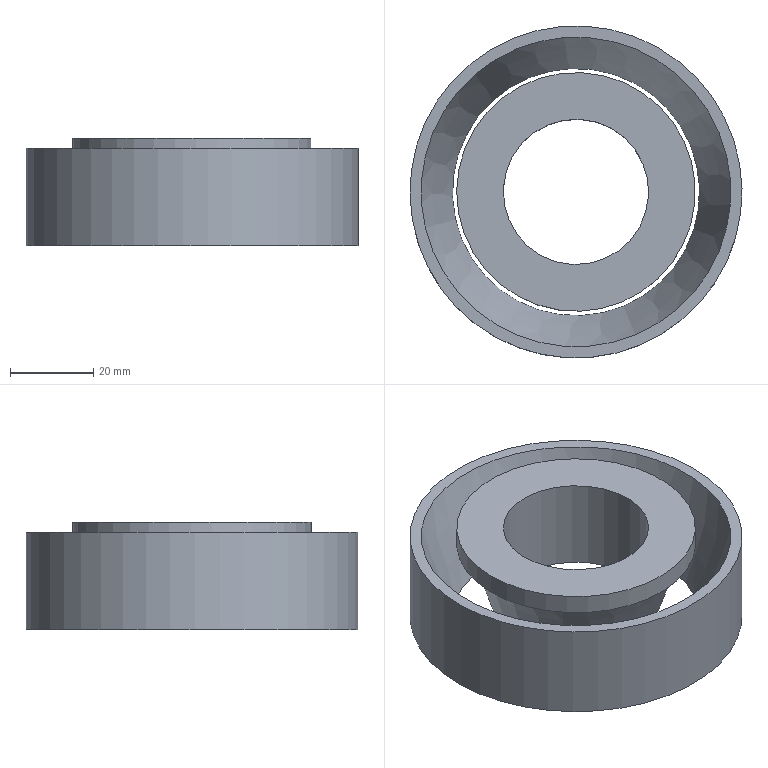Component | NX | GUNZIZHOUCHOU | 2 solids | 10 faces | box 80 x 80 x 26 mm | volume 55024 mm3 | plane 5 | cylinder 3 | cone 2 | commonest cylinder face diameters 35 x1 57.5 x1 80 x1
STEP:
#1=CARTESIAN_POINT('',(0.,0.,0.));
#2=DIRECTION('',(0.,0.,1.));
#3=DIRECTION('',(1.,0.,0.));
#4=AXIS2_PLACEMENT_3D('',#1,#2,#3);
#5=CARTESIAN_POINT('',(6.703,-16.165,0.45));
#6=VERTEX_POINT('',#5);
#7=CARTESIAN_POINT('',(0.,0.,0.45));
#8=DIRECTION('',(0.,0.,1.));
#9=DIRECTION('',(0.383,-0.9237,0.));
#10=AXIS2_PLACEMENT_3D('',#7,#8,#9);
#11=CIRCLE('',#10,17.5);
#12=CARTESIAN_POINT('',(18.43,7.643,0.45));
#13=DIRECTION('',(0.,0.,-1.));
#14=DIRECTION('',(-0.383,0.9237,0.));
#15=AXIS2_PLACEMENT_3D('',#12,#13,#14);
#16=PLANE('',#15);
#17=CARTESIAN_POINT('',(-17.5,-19.952));
#18=CARTESIAN_POINT('',(-17.5,10.359));
#19=CARTESIAN_POINT('',(8.75,-4.797));
#20=CARTESIAN_POINT('',(35.,-19.952));
#21=CARTESIAN_POINT('',(8.75,-35.107));
#22=CARTESIAN_POINT('',(-17.5,-50.263));
#23=CARTESIAN_POINT('',(-17.5,-19.952));
#24=(BOUNDED_CURVE()B_SPLINE_CURVE(2,(#17,#18,#19,#20,#21,#22,#23),.UNSPECIFIED.,.T.,.F.)B_SPLINE_CURVE_WITH_KNOTS((1,2,2,2,2,1),(-2.094,0.,2.094,4.189,6.283,8.378),.UNSPECIFIED.)CURVE()GEOMETRIC_REPRESENTATION_ITEM()RATIONAL_B_SPLINE_CURVE((1.,0.5,1.,0.5,1.,0.5,1.))REPRESENTATION_ITEM(''));
#25=(GEOMETRIC_REPRESENTATION_CONTEXT(2)PARAMETRIC_REPRESENTATION_CONTEXT()REPRESENTATION_CONTEXT('',''));
#26=DEFINITIONAL_REPRESENTATION('',(#24),#25);
#27=PCURVE('',#16,#26);
#28=CARTESIAN_POINT('',(0.,0.,23.));
#29=DIRECTION('',(0.,0.,1.));
#30=DIRECTION('',(0.383,-0.9237,0.));
#31=AXIS2_PLACEMENT_3D('',#28,#29,#30);
#32=CYLINDRICAL_SURFACE('',#31,17.5);
#33=CARTESIAN_POINT('',(0.,-22.55));
#34=DIRECTION('',(1.,0.));
#35=VECTOR('',#34,1.);
#36=LINE('',#33,#35);
#37=(GEOMETRIC_REPRESENTATION_CONTEXT(2)PARAMETRIC_REPRESENTATION_CONTEXT()REPRESENTATION_CONTEXT('',''));
#38=DEFINITIONAL_REPRESENTATION('',(#36),#37);
#39=PCURVE('',#32,#38);
#40=SURFACE_CURVE('',#11,(#27,#39),.PCURVE_S1.);
#41=EDGE_CURVE('',#6,#6,#40,.T.);
#42=ORIENTED_EDGE('',*,*,#41,.T.);
#43=EDGE_LOOP('',(#42));
#44=FACE_BOUND('',#43,.T.);
#45=CARTESIAN_POINT('',(7.643,-18.43,0.45));
#46=VERTEX_POINT('',#45);
#47=CARTESIAN_POINT('',(0.,0.,0.45));
#48=DIRECTION('',(0.,0.,1.));
#49=DIRECTION('',(0.383,-0.9237,0.));
#50=AXIS2_PLACEMENT_3D('',#47,#48,#49);
#51=CIRCLE('',#50,19.952);
#52=CARTESIAN_POINT('',(-19.952,-19.952));
#53=CARTESIAN_POINT('',(-19.952,14.606));
#54=CARTESIAN_POINT('',(9.976,-2.673));
#55=CARTESIAN_POINT('',(39.904,-19.952));
#56=CARTESIAN_POINT('',(9.976,-37.231));
#57=CARTESIAN_POINT('',(-19.952,-54.51));
#58=CARTESIAN_POINT('',(-19.952,-19.952));
#59=(BOUNDED_CURVE()B_SPLINE_CURVE(2,(#52,#53,#54,#55,#56,#57,#58),.UNSPECIFIED.,.T.,.F.)B_SPLINE_CURVE_WITH_KNOTS((1,2,2,2,2,1),(-2.094,0.,2.094,4.189,6.283,8.378),.UNSPECIFIED.)CURVE()GEOMETRIC_REPRESENTATION_ITEM()RATIONAL_B_SPLINE_CURVE((1.,0.5,1.,0.5,1.,0.5,1.))REPRESENTATION_ITEM(''));
#60=(GEOMETRIC_REPRESENTATION_CONTEXT(2)PARAMETRIC_REPRESENTATION_CONTEXT()REPRESENTATION_CONTEXT('',''));
#61=DEFINITIONAL_REPRESENTATION('',(#59),#60);
#62=PCURVE('',#16,#61);
#63=CARTESIAN_POINT('',(0.,0.,18.25));
#64=DIRECTION('',(0.,0.,1.));
#65=DIRECTION('',(0.383,-0.9237,0.));
#66=AXIS2_PLACEMENT_3D('',#63,#64,#65);
#67=CONICAL_SURFACE('',#66,25.952,0.3251);
#68=CARTESIAN_POINT('',(0.,-17.8));
#69=DIRECTION('',(1.,0.));
#70=VECTOR('',#69,1.);
#71=LINE('',#68,#70);
#72=(GEOMETRIC_REPRESENTATION_CONTEXT(2)PARAMETRIC_REPRESENTATION_CONTEXT()REPRESENTATION_CONTEXT('',''));
#73=DEFINITIONAL_REPRESENTATION('',(#71),#72);
#74=PCURVE('',#67,#73);
#75=SURFACE_CURVE('',#51,(#62,#74),.PCURVE_S1.);
#76=EDGE_CURVE('',#46,#46,#75,.T.);
#77=ORIENTED_EDGE('',*,*,#76,.F.);
#78=EDGE_LOOP('',(#77));
#79=FACE_BOUND('',#78,.T.);
#80=ADVANCED_FACE('',(#44,#79),#16,.T.);
#81=CARTESIAN_POINT('',(6.703,-16.165,23.));
#82=VERTEX_POINT('',#81);
#83=CARTESIAN_POINT('',(0.,0.,23.));
#84=DIRECTION('',(0.,0.,1.));
#85=DIRECTION('',(0.383,-0.9237,0.));
#86=AXIS2_PLACEMENT_3D('',#83,#84,#85);
#87=CIRCLE('',#86,17.5);
#88=CARTESIAN_POINT('',(0.,0.));
#89=DIRECTION('',(1.,0.));
#90=VECTOR('',#89,1.);
#91=LINE('',#88,#90);
#92=(GEOMETRIC_REPRESENTATION_CONTEXT(2)PARAMETRIC_REPRESENTATION_CONTEXT()REPRESENTATION_CONTEXT('',''));
#93=DEFINITIONAL_REPRESENTATION('',(#91),#92);
#94=PCURVE('',#32,#93);
#95=CARTESIAN_POINT('',(16.165,6.703,23.));
#96=DIRECTION('',(0.,0.,1.));
#97=DIRECTION('',(0.383,-0.9237,0.));
#98=AXIS2_PLACEMENT_3D('',#95,#96,#97);
#99=PLANE('',#98);
#100=CARTESIAN_POINT('',(-0.,-17.5));
#101=DIRECTION('',(1.,0.));
#102=AXIS2_PLACEMENT_2D('',#100,#101);
#103=CIRCLE('',#102,17.5);
#104=(GEOMETRIC_REPRESENTATION_CONTEXT(2)PARAMETRIC_REPRESENTATION_CONTEXT()REPRESENTATION_CONTEXT('',''));
#105=DEFINITIONAL_REPRESENTATION('',(#103),#104);
#106=PCURVE('',#99,#105);
#107=SURFACE_CURVE('',#87,(#94,#106),.PCURVE_S1.);
#108=EDGE_CURVE('',#82,#82,#107,.T.);
#109=ORIENTED_EDGE('',*,*,#108,.F.);
#110=CARTESIAN_POINT('',(6.703,-16.165,0.45));
#111=CARTESIAN_POINT('',(6.703,-16.165,23.));
#112=B_SPLINE_CURVE_WITH_KNOTS('',1,(#110,#111),.UNSPECIFIED.,.F.,.F.,(2,2),(-22.55,0.),.PIECEWISE_BEZIER_KNOTS.);
#113=CARTESIAN_POINT('',(0.,0.));
#114=DIRECTION('',(0.,1.));
#115=VECTOR('',#114,1.);
#116=LINE('',#113,#115);
#117=(GEOMETRIC_REPRESENTATION_CONTEXT(2)PARAMETRIC_REPRESENTATION_CONTEXT()REPRESENTATION_CONTEXT('',''));
#118=DEFINITIONAL_REPRESENTATION('',(#116),#117);
#119=PCURVE('',#32,#118);
#120=CARTESIAN_POINT('',(6.283,0.));
#121=DIRECTION('',(0.,1.));
#122=VECTOR('',#121,1.);
#123=LINE('',#120,#122);
#124=(GEOMETRIC_REPRESENTATION_CONTEXT(2)PARAMETRIC_REPRESENTATION_CONTEXT()REPRESENTATION_CONTEXT('',''));
#125=DEFINITIONAL_REPRESENTATION('',(#123),#124);
#126=PCURVE('',#32,#125);
#127=SEAM_CURVE('',#112,(#119,#126),.PCURVE_S1.);
#128=EDGE_CURVE('',#6,#82,#127,.T.);
#129=ORIENTED_EDGE('',*,*,#128,.F.);
#130=ORIENTED_EDGE('',*,*,#41,.T.);
#131=ORIENTED_EDGE('',*,*,#128,.T.);
#132=EDGE_LOOP('',(#109,#129,#130,#131));
#133=FACE_BOUND('',#132,.F.);
#134=ADVANCED_FACE('',(#133),#32,.F.);
#135=CARTESIAN_POINT('',(11.013,-26.557,23.));
#136=VERTEX_POINT('',#135);
#137=CARTESIAN_POINT('',(0.,0.,23.));
#138=DIRECTION('',(0.,0.,1.));
#139=DIRECTION('',(0.383,-0.9237,0.));
#140=AXIS2_PLACEMENT_3D('',#137,#138,#139);
#141=CIRCLE('',#140,28.75);
#142=CARTESIAN_POINT('',(-0.,-17.5));
#143=DIRECTION('',(1.,0.));
#144=AXIS2_PLACEMENT_2D('',#142,#143);
#145=CIRCLE('',#144,28.75);
#146=(GEOMETRIC_REPRESENTATION_CONTEXT(2)PARAMETRIC_REPRESENTATION_CONTEXT()REPRESENTATION_CONTEXT('',''));
#147=DEFINITIONAL_REPRESENTATION('',(#145),#146);
#148=PCURVE('',#99,#147);
#149=CARTESIAN_POINT('',(0.,0.,23.));
#150=DIRECTION('',(0.,0.,1.));
#151=DIRECTION('',(0.383,-0.9237,0.));
#152=AXIS2_PLACEMENT_3D('',#149,#150,#151);
#153=CYLINDRICAL_SURFACE('',#152,28.75);
#154=CARTESIAN_POINT('',(0.,0.));
#155=DIRECTION('',(1.,0.));
#156=VECTOR('',#155,1.);
#157=LINE('',#154,#156);
#158=(GEOMETRIC_REPRESENTATION_CONTEXT(2)PARAMETRIC_REPRESENTATION_CONTEXT()REPRESENTATION_CONTEXT('',''));
#159=DEFINITIONAL_REPRESENTATION('',(#157),#158);
#160=PCURVE('',#153,#159);
#161=SURFACE_CURVE('',#141,(#148,#160),.PCURVE_S1.);
#162=EDGE_CURVE('',#136,#136,#161,.T.);
#163=ORIENTED_EDGE('',*,*,#162,.T.);
#164=EDGE_LOOP('',(#163));
#165=FACE_BOUND('',#164,.T.);
#166=ORIENTED_EDGE('',*,*,#108,.F.);
#167=EDGE_LOOP('',(#166));
#168=FACE_BOUND('',#167,.T.);
#169=ADVANCED_FACE('',(#165,#168),#99,.T.);
#170=CARTESIAN_POINT('',(11.013,-26.557,18.25));
#171=VERTEX_POINT('',#170);
#172=CARTESIAN_POINT('',(0.,0.,18.25));
#173=DIRECTION('',(0.,0.,1.));
#174=DIRECTION('',(0.383,-0.9237,0.));
#175=AXIS2_PLACEMENT_3D('',#172,#173,#174);
#176=CIRCLE('',#175,28.75);
#177=CARTESIAN_POINT('',(0.,-4.75));
#178=DIRECTION('',(1.,0.));
#179=VECTOR('',#178,1.);
#180=LINE('',#177,#179);
#181=(GEOMETRIC_REPRESENTATION_CONTEXT(2)PARAMETRIC_REPRESENTATION_CONTEXT()REPRESENTATION_CONTEXT('',''));
#182=DEFINITIONAL_REPRESENTATION('',(#180),#181);
#183=PCURVE('',#153,#182);
#184=CARTESIAN_POINT('',(26.557,11.013,18.25));
#185=DIRECTION('',(0.,0.,-1.));
#186=DIRECTION('',(-0.383,0.9237,0.));
#187=AXIS2_PLACEMENT_3D('',#184,#185,#186);
#188=PLANE('',#187);
#189=CARTESIAN_POINT('',(-28.75,-28.75));
#190=CARTESIAN_POINT('',(-28.75,21.046));
#191=CARTESIAN_POINT('',(14.375,-3.852));
#192=CARTESIAN_POINT('',(57.5,-28.75));
#193=CARTESIAN_POINT('',(14.375,-53.648));
#194=CARTESIAN_POINT('',(-28.75,-78.546));
#195=CARTESIAN_POINT('',(-28.75,-28.75));
#196=(BOUNDED_CURVE()B_SPLINE_CURVE(2,(#189,#190,#191,#192,#193,#194,#195),.UNSPECIFIED.,.T.,.F.)B_SPLINE_CURVE_WITH_KNOTS((1,2,2,2,2,1),(-2.094,0.,2.094,4.189,6.283,8.378),.UNSPECIFIED.)CURVE()GEOMETRIC_REPRESENTATION_ITEM()RATIONAL_B_SPLINE_CURVE((1.,0.5,1.,0.5,1.,0.5,1.))REPRESENTATION_ITEM(''));
#197=(GEOMETRIC_REPRESENTATION_CONTEXT(2)PARAMETRIC_REPRESENTATION_CONTEXT()REPRESENTATION_CONTEXT('',''));
#198=DEFINITIONAL_REPRESENTATION('',(#196),#197);
#199=PCURVE('',#188,#198);
#200=SURFACE_CURVE('',#176,(#183,#199),.PCURVE_S1.);
#201=EDGE_CURVE('',#171,#171,#200,.T.);
#202=ORIENTED_EDGE('',*,*,#201,.T.);
#203=CARTESIAN_POINT('',(11.013,-26.557,18.25));
#204=CARTESIAN_POINT('',(11.013,-26.557,23.));
#205=B_SPLINE_CURVE_WITH_KNOTS('',1,(#203,#204),.UNSPECIFIED.,.F.,.F.,(2,2),(-4.75,0.),.PIECEWISE_BEZIER_KNOTS.);
#206=CARTESIAN_POINT('',(6.283,0.));
#207=DIRECTION('',(0.,1.));
#208=VECTOR('',#207,1.);
#209=LINE('',#206,#208);
#210=(GEOMETRIC_REPRESENTATION_CONTEXT(2)PARAMETRIC_REPRESENTATION_CONTEXT()REPRESENTATION_CONTEXT('',''));
#211=DEFINITIONAL_REPRESENTATION('',(#209),#210);
#212=PCURVE('',#153,#211);
#213=CARTESIAN_POINT('',(0.,0.));
#214=DIRECTION('',(0.,1.));
#215=VECTOR('',#214,1.);
#216=LINE('',#213,#215);
#217=(GEOMETRIC_REPRESENTATION_CONTEXT(2)PARAMETRIC_REPRESENTATION_CONTEXT()REPRESENTATION_CONTEXT('',''));
#218=DEFINITIONAL_REPRESENTATION('',(#216),#217);
#219=PCURVE('',#153,#218);
#220=SEAM_CURVE('',#205,(#212,#219),.PCURVE_S1.);
#221=EDGE_CURVE('',#171,#136,#220,.T.);
#222=ORIENTED_EDGE('',*,*,#221,.T.);
#223=ORIENTED_EDGE('',*,*,#162,.F.);
#224=ORIENTED_EDGE('',*,*,#221,.F.);
#225=EDGE_LOOP('',(#202,#222,#223,#224));
#226=FACE_BOUND('',#225,.T.);
#227=ADVANCED_FACE('',(#226),#153,.T.);
#228=CARTESIAN_POINT('',(9.941,-23.973,18.25));
#229=VERTEX_POINT('',#228);
#230=CARTESIAN_POINT('',(0.,0.,18.25));
#231=DIRECTION('',(0.,0.,1.));
#232=DIRECTION('',(0.383,-0.9237,0.));
#233=AXIS2_PLACEMENT_3D('',#230,#231,#232);
#234=CIRCLE('',#233,25.952);
#235=CARTESIAN_POINT('',(-25.952,-28.75));
#236=CARTESIAN_POINT('',(-25.952,16.2));
#237=CARTESIAN_POINT('',(12.976,-6.275));
#238=CARTESIAN_POINT('',(51.904,-28.75));
#239=CARTESIAN_POINT('',(12.976,-51.225));
#240=CARTESIAN_POINT('',(-25.952,-73.7));
#241=CARTESIAN_POINT('',(-25.952,-28.75));
#242=(BOUNDED_CURVE()B_SPLINE_CURVE(2,(#235,#236,#237,#238,#239,#240,#241),.UNSPECIFIED.,.T.,.F.)B_SPLINE_CURVE_WITH_KNOTS((1,2,2,2,2,1),(-2.094,0.,2.094,4.189,6.283,8.378),.UNSPECIFIED.)CURVE()GEOMETRIC_REPRESENTATION_ITEM()RATIONAL_B_SPLINE_CURVE((1.,0.5,1.,0.5,1.,0.5,1.))REPRESENTATION_ITEM(''));
#243=(GEOMETRIC_REPRESENTATION_CONTEXT(2)PARAMETRIC_REPRESENTATION_CONTEXT()REPRESENTATION_CONTEXT('',''));
#244=DEFINITIONAL_REPRESENTATION('',(#242),#243);
#245=PCURVE('',#188,#244);
#246=CARTESIAN_POINT('',(0.,0.));
#247=DIRECTION('',(1.,-0.));
#248=VECTOR('',#247,1.);
#249=LINE('',#246,#248);
#250=(GEOMETRIC_REPRESENTATION_CONTEXT(2)PARAMETRIC_REPRESENTATION_CONTEXT()REPRESENTATION_CONTEXT('',''));
#251=DEFINITIONAL_REPRESENTATION('',(#249),#250);
#252=PCURVE('',#67,#251);
#253=SURFACE_CURVE('',#234,(#245,#252),.PCURVE_S1.);
#254=EDGE_CURVE('',#229,#229,#253,.T.);
#255=ORIENTED_EDGE('',*,*,#254,.T.);
#256=EDGE_LOOP('',(#255));
#257=FACE_BOUND('',#256,.T.);
#258=ORIENTED_EDGE('',*,*,#201,.F.);
#259=EDGE_LOOP('',(#258));
#260=FACE_BOUND('',#259,.T.);
#261=ADVANCED_FACE('',(#257,#260),#188,.T.);
#262=ORIENTED_EDGE('',*,*,#76,.T.);
#263=CARTESIAN_POINT('',(7.643,-18.43,0.45));
#264=CARTESIAN_POINT('',(9.941,-23.973,18.25));
#265=B_SPLINE_CURVE_WITH_KNOTS('',1,(#263,#264),.UNSPECIFIED.,.F.,.F.,(2,2),(-18.784,0.),.PIECEWISE_BEZIER_KNOTS.);
#266=CARTESIAN_POINT('',(6.283,0.));
#267=DIRECTION('',(0.,1.));
#268=VECTOR('',#267,1.);
#269=LINE('',#266,#268);
#270=(GEOMETRIC_REPRESENTATION_CONTEXT(2)PARAMETRIC_REPRESENTATION_CONTEXT()REPRESENTATION_CONTEXT('',''));
#271=DEFINITIONAL_REPRESENTATION('',(#269),#270);
#272=PCURVE('',#67,#271);
#273=CARTESIAN_POINT('',(0.,0.));
#274=DIRECTION('',(0.,1.));
#275=VECTOR('',#274,1.);
#276=LINE('',#273,#275);
#277=(GEOMETRIC_REPRESENTATION_CONTEXT(2)PARAMETRIC_REPRESENTATION_CONTEXT()REPRESENTATION_CONTEXT('',''));
#278=DEFINITIONAL_REPRESENTATION('',(#276),#277);
#279=PCURVE('',#67,#278);
#280=SEAM_CURVE('',#265,(#272,#279),.PCURVE_S1.);
#281=EDGE_CURVE('',#46,#229,#280,.T.);
#282=ORIENTED_EDGE('',*,*,#281,.T.);
#283=ORIENTED_EDGE('',*,*,#254,.F.);
#284=ORIENTED_EDGE('',*,*,#281,.F.);
#285=EDGE_LOOP('',(#262,#282,#283,#284));
#286=FACE_BOUND('',#285,.T.);
#287=ADVANCED_FACE('',(#286),#67,.T.);
#288=CLOSED_SHELL('',(#80,#134,#169,#227,#261,#287));
#289=MANIFOLD_SOLID_BREP('',#288);
#290=(LENGTH_UNIT()NAMED_UNIT(*)SI_UNIT(.MILLI.,.METRE.));
#291=UNCERTAINTY_MEASURE_WITH_UNIT(LENGTH_MEASURE(0.00001),#290,'','');
#292=(NAMED_UNIT(*)PLANE_ANGLE_UNIT()SI_UNIT($,.RADIAN.));
#293=(NAMED_UNIT(*)SI_UNIT($,.STERADIAN.)SOLID_ANGLE_UNIT());
#294=(GEOMETRIC_REPRESENTATION_CONTEXT(3)GLOBAL_UNCERTAINTY_ASSIGNED_CONTEXT((#291))GLOBAL_UNIT_ASSIGNED_CONTEXT((#290,#292,#293))REPRESENTATION_CONTEXT('',''));
#295=ADVANCED_BREP_SHAPE_REPRESENTATION('',(#4,#289),#294);
#296=CARTESIAN_POINT('',(0.,0.,0.));
#297=DIRECTION('',(0.,0.,1.));
#298=DIRECTION('',(1.,0.,0.));
#299=AXIS2_PLACEMENT_3D('',#296,#297,#298);
#300=CARTESIAN_POINT('',(0.,0.,0.));
#301=DIRECTION('',(0.,0.,1.));
#302=DIRECTION('',(1.,0.,0.));
#303=AXIS2_PLACEMENT_3D('',#300,#301,#302);
#304=(LENGTH_UNIT()NAMED_UNIT(*)SI_UNIT(.MILLI.,.METRE.));
#305=UNCERTAINTY_MEASURE_WITH_UNIT(LENGTH_MEASURE(0.00001),#304,'','');
#306=(NAMED_UNIT(*)PLANE_ANGLE_UNIT()SI_UNIT($,.RADIAN.));
#307=(NAMED_UNIT(*)SI_UNIT($,.STERADIAN.)SOLID_ANGLE_UNIT());
#308=(GEOMETRIC_REPRESENTATION_CONTEXT(3)GLOBAL_UNCERTAINTY_ASSIGNED_CONTEXT((#305))GLOBAL_UNIT_ASSIGNED_CONTEXT((#304,#306,#307))REPRESENTATION_CONTEXT('',''));
#309=SHAPE_REPRESENTATION('',(#4,#299,#303),#308);
#310=ITEM_DEFINED_TRANSFORMATION('','',#4,#299);
#311=(REPRESENTATION_RELATIONSHIP('','',#295,#309)REPRESENTATION_RELATIONSHIP_WITH_TRANSFORMATION(#310)SHAPE_REPRESENTATION_RELATIONSHIP());
#312=CARTESIAN_POINT('',(15.322,-36.949,20.5));
#313=VERTEX_POINT('',#312);
#314=CARTESIAN_POINT('',(0.,0.,20.5));
#315=DIRECTION('',(0.,0.,1.));
#316=DIRECTION('',(0.383,-0.9237,0.));
#317=AXIS2_PLACEMENT_3D('',#314,#315,#316);
#318=CIRCLE('',#317,40.);
#319=CARTESIAN_POINT('',(0.,0.,23.));
#320=DIRECTION('',(0.,0.,1.));
#321=DIRECTION('',(0.383,-0.9237,0.));
#322=AXIS2_PLACEMENT_3D('',#319,#320,#321);
#323=CYLINDRICAL_SURFACE('',#322,40.);
#324=CARTESIAN_POINT('',(0.,-2.5));
#325=DIRECTION('',(1.,0.));
#326=VECTOR('',#325,1.);
#327=LINE('',#324,#326);
#328=(GEOMETRIC_REPRESENTATION_CONTEXT(2)PARAMETRIC_REPRESENTATION_CONTEXT()REPRESENTATION_CONTEXT('',''));
#329=DEFINITIONAL_REPRESENTATION('',(#327),#328);
#330=PCURVE('',#323,#329);
#331=CARTESIAN_POINT('',(-15.322,36.949,20.5));
#332=DIRECTION('',(0.,0.,-1.));
#333=DIRECTION('',(-0.383,0.9237,0.));
#334=AXIS2_PLACEMENT_3D('',#331,#332,#333);
#335=PLANE('',#334);
#336=CARTESIAN_POINT('',(-80.,-0.));
#337=CARTESIAN_POINT('',(-80.,69.282));
#338=CARTESIAN_POINT('',(-20.,34.641));
#339=CARTESIAN_POINT('',(40.,-0.));
#340=CARTESIAN_POINT('',(-20.,-34.641));
#341=CARTESIAN_POINT('',(-80.,-69.282));
#342=CARTESIAN_POINT('',(-80.,-0.));
#343=(BOUNDED_CURVE()B_SPLINE_CURVE(2,(#336,#337,#338,#339,#340,#341,#342),.UNSPECIFIED.,.T.,.F.)B_SPLINE_CURVE_WITH_KNOTS((1,2,2,2,2,1),(-2.094,0.,2.094,4.189,6.283,8.378),.UNSPECIFIED.)CURVE()GEOMETRIC_REPRESENTATION_ITEM()RATIONAL_B_SPLINE_CURVE((1.,0.5,1.,0.5,1.,0.5,1.))REPRESENTATION_ITEM(''));
#344=(GEOMETRIC_REPRESENTATION_CONTEXT(2)PARAMETRIC_REPRESENTATION_CONTEXT()REPRESENTATION_CONTEXT('',''));
#345=DEFINITIONAL_REPRESENTATION('',(#343),#344);
#346=PCURVE('',#335,#345);
#347=SURFACE_CURVE('',#318,(#330,#346),.PCURVE_S1.);
#348=EDGE_CURVE('',#313,#313,#347,.T.);
#349=ORIENTED_EDGE('',*,*,#348,.F.);
#350=CARTESIAN_POINT('',(15.322,-36.949,-3.));
#351=VERTEX_POINT('',#350);
#352=CARTESIAN_POINT('',(15.322,-36.949,-3.));
#353=CARTESIAN_POINT('',(15.322,-36.949,20.5));
#354=B_SPLINE_CURVE_WITH_KNOTS('',1,(#352,#353),.UNSPECIFIED.,.F.,.F.,(2,2),(-26.,-2.5),.PIECEWISE_BEZIER_KNOTS.);
#355=CARTESIAN_POINT('',(0.,0.));
#356=DIRECTION('',(0.,1.));
#357=VECTOR('',#356,1.);
#358=LINE('',#355,#357);
#359=(GEOMETRIC_REPRESENTATION_CONTEXT(2)PARAMETRIC_REPRESENTATION_CONTEXT()REPRESENTATION_CONTEXT('',''));
#360=DEFINITIONAL_REPRESENTATION('',(#358),#359);
#361=PCURVE('',#323,#360);
#362=CARTESIAN_POINT('',(6.283,0.));
#363=DIRECTION('',(0.,1.));
#364=VECTOR('',#363,1.);
#365=LINE('',#362,#364);
#366=(GEOMETRIC_REPRESENTATION_CONTEXT(2)PARAMETRIC_REPRESENTATION_CONTEXT()REPRESENTATION_CONTEXT('',''));
#367=DEFINITIONAL_REPRESENTATION('',(#365),#366);
#368=PCURVE('',#323,#367);
#369=SEAM_CURVE('',#354,(#361,#368),.PCURVE_S1.);
#370=EDGE_CURVE('',#351,#313,#369,.T.);
#371=ORIENTED_EDGE('',*,*,#370,.F.);
#372=CARTESIAN_POINT('',(0.,0.,-3.));
#373=DIRECTION('',(0.,0.,1.));
#374=DIRECTION('',(0.383,-0.9237,0.));
#375=AXIS2_PLACEMENT_3D('',#372,#373,#374);
#376=CIRCLE('',#375,40.);
#377=CARTESIAN_POINT('',(0.,-26.));
#378=DIRECTION('',(1.,0.));
#379=VECTOR('',#378,1.);
#380=LINE('',#377,#379);
#381=(GEOMETRIC_REPRESENTATION_CONTEXT(2)PARAMETRIC_REPRESENTATION_CONTEXT()REPRESENTATION_CONTEXT('',''));
#382=DEFINITIONAL_REPRESENTATION('',(#380),#381);
#383=PCURVE('',#323,#382);
#384=CARTESIAN_POINT('',(-11.402,27.496,-3.));
#385=DIRECTION('',(0.,0.,1.));
#386=DIRECTION('',(0.383,-0.9237,0.));
#387=AXIS2_PLACEMENT_3D('',#384,#385,#386);
#388=PLANE('',#387);
#389=CARTESIAN_POINT('',(29.766,0.));
#390=DIRECTION('',(1.,0.));
#391=AXIS2_PLACEMENT_2D('',#389,#390);
#392=CIRCLE('',#391,40.);
#393=(GEOMETRIC_REPRESENTATION_CONTEXT(2)PARAMETRIC_REPRESENTATION_CONTEXT()REPRESENTATION_CONTEXT('',''));
#394=DEFINITIONAL_REPRESENTATION('',(#392),#393);
#395=PCURVE('',#388,#394);
#396=SURFACE_CURVE('',#376,(#383,#395),.PCURVE_S1.);
#397=EDGE_CURVE('',#351,#351,#396,.T.);
#398=ORIENTED_EDGE('',*,*,#397,.T.);
#399=ORIENTED_EDGE('',*,*,#370,.T.);
#400=EDGE_LOOP('',(#349,#371,#398,#399));
#401=FACE_BOUND('',#400,.T.);
#402=ADVANCED_FACE('',(#401),#323,.T.);
#403=CARTESIAN_POINT('',(14.288,-34.455,20.5));
#404=VERTEX_POINT('',#403);
#405=CARTESIAN_POINT('',(0.,0.,20.5));
#406=DIRECTION('',(0.,0.,1.));
#407=DIRECTION('',(0.383,-0.9237,0.));
#408=AXIS2_PLACEMENT_3D('',#405,#406,#407);
#409=CIRCLE('',#408,37.3);
#410=CARTESIAN_POINT('',(-77.3,-0.));
#411=CARTESIAN_POINT('',(-77.3,64.605));
#412=CARTESIAN_POINT('',(-21.35,32.303));
#413=CARTESIAN_POINT('',(34.6,-0.));
#414=CARTESIAN_POINT('',(-21.35,-32.303));
#415=CARTESIAN_POINT('',(-77.3,-64.605));
#416=CARTESIAN_POINT('',(-77.3,-0.));
#417=(BOUNDED_CURVE()B_SPLINE_CURVE(2,(#410,#411,#412,#413,#414,#415,#416),.UNSPECIFIED.,.T.,.F.)B_SPLINE_CURVE_WITH_KNOTS((1,2,2,2,2,1),(-2.094,0.,2.094,4.189,6.283,8.378),.UNSPECIFIED.)CURVE()GEOMETRIC_REPRESENTATION_ITEM()RATIONAL_B_SPLINE_CURVE((1.,0.5,1.,0.5,1.,0.5,1.))REPRESENTATION_ITEM(''));
#418=(GEOMETRIC_REPRESENTATION_CONTEXT(2)PARAMETRIC_REPRESENTATION_CONTEXT()REPRESENTATION_CONTEXT('',''));
#419=DEFINITIONAL_REPRESENTATION('',(#417),#418);
#420=PCURVE('',#335,#419);
#421=CARTESIAN_POINT('',(0.,0.,20.5));
#422=DIRECTION('',(0.,0.,1.));
#423=DIRECTION('',(0.383,-0.9237,0.));
#424=AXIS2_PLACEMENT_3D('',#421,#422,#423);
#425=CONICAL_SURFACE('',#424,37.3,0.3102);
#426=CARTESIAN_POINT('',(0.,0.));
#427=DIRECTION('',(1.,0.));
#428=VECTOR('',#427,1.);
#429=LINE('',#426,#428);
#430=(GEOMETRIC_REPRESENTATION_CONTEXT(2)PARAMETRIC_REPRESENTATION_CONTEXT()REPRESENTATION_CONTEXT('',''));
#431=DEFINITIONAL_REPRESENTATION('',(#429),#430);
#432=PCURVE('',#425,#431);
#433=SURFACE_CURVE('',#409,(#420,#432),.PCURVE_S1.);
#434=EDGE_CURVE('',#404,#404,#433,.T.);
#435=ORIENTED_EDGE('',*,*,#434,.F.);
#436=EDGE_LOOP('',(#435));
#437=FACE_BOUND('',#436,.T.);
#438=ORIENTED_EDGE('',*,*,#348,.T.);
#439=EDGE_LOOP('',(#438));
#440=FACE_BOUND('',#439,.T.);
#441=ADVANCED_FACE('',(#437,#440),#335,.F.);
#442=CARTESIAN_POINT('',(11.402,-27.496,-3.));
#443=VERTEX_POINT('',#442);
#444=CARTESIAN_POINT('',(0.,0.,-3.));
#445=DIRECTION('',(0.,0.,1.));
#446=DIRECTION('',(0.383,-0.9237,0.));
#447=AXIS2_PLACEMENT_3D('',#444,#445,#446);
#448=CIRCLE('',#447,29.766);
#449=CARTESIAN_POINT('',(0.,-23.5));
#450=DIRECTION('',(1.,0.));
#451=VECTOR('',#450,1.);
#452=LINE('',#449,#451);
#453=(GEOMETRIC_REPRESENTATION_CONTEXT(2)PARAMETRIC_REPRESENTATION_CONTEXT()REPRESENTATION_CONTEXT('',''));
#454=DEFINITIONAL_REPRESENTATION('',(#452),#453);
#455=PCURVE('',#425,#454);
#456=CARTESIAN_POINT('',(29.766,0.));
#457=DIRECTION('',(1.,0.));
#458=AXIS2_PLACEMENT_2D('',#456,#457);
#459=CIRCLE('',#458,29.766);
#460=(GEOMETRIC_REPRESENTATION_CONTEXT(2)PARAMETRIC_REPRESENTATION_CONTEXT()REPRESENTATION_CONTEXT('',''));
#461=DEFINITIONAL_REPRESENTATION('',(#459),#460);
#462=PCURVE('',#388,#461);
#463=SURFACE_CURVE('',#448,(#455,#462),.PCURVE_S1.);
#464=EDGE_CURVE('',#443,#443,#463,.T.);
#465=ORIENTED_EDGE('',*,*,#464,.T.);
#466=CARTESIAN_POINT('',(11.402,-27.496,-3.));
#467=CARTESIAN_POINT('',(14.288,-34.455,20.5));
#468=B_SPLINE_CURVE_WITH_KNOTS('',1,(#466,#467),.UNSPECIFIED.,.F.,.F.,(2,2),(-24.678,0.),.PIECEWISE_BEZIER_KNOTS.);
#469=CARTESIAN_POINT('',(6.283,0.));
#470=DIRECTION('',(0.,1.));
#471=VECTOR('',#470,1.);
#472=LINE('',#469,#471);
#473=(GEOMETRIC_REPRESENTATION_CONTEXT(2)PARAMETRIC_REPRESENTATION_CONTEXT()REPRESENTATION_CONTEXT('',''));
#474=DEFINITIONAL_REPRESENTATION('',(#472),#473);
#475=PCURVE('',#425,#474);
#476=CARTESIAN_POINT('',(0.,0.));
#477=DIRECTION('',(0.,1.));
#478=VECTOR('',#477,1.);
#479=LINE('',#476,#478);
#480=(GEOMETRIC_REPRESENTATION_CONTEXT(2)PARAMETRIC_REPRESENTATION_CONTEXT()REPRESENTATION_CONTEXT('',''));
#481=DEFINITIONAL_REPRESENTATION('',(#479),#480);
#482=PCURVE('',#425,#481);
#483=SEAM_CURVE('',#468,(#475,#482),.PCURVE_S1.);
#484=EDGE_CURVE('',#443,#404,#483,.T.);
#485=ORIENTED_EDGE('',*,*,#484,.T.);
#486=ORIENTED_EDGE('',*,*,#434,.F.);
#487=ORIENTED_EDGE('',*,*,#484,.F.);
#488=EDGE_LOOP('',(#465,#485,#486,#487));
#489=FACE_BOUND('',#488,.F.);
#490=ADVANCED_FACE('',(#489),#425,.F.);
#491=ORIENTED_EDGE('',*,*,#397,.F.);
#492=EDGE_LOOP('',(#491));
#493=FACE_BOUND('',#492,.T.);
#494=ORIENTED_EDGE('',*,*,#464,.T.);
#495=EDGE_LOOP('',(#494));
#496=FACE_BOUND('',#495,.T.);
#497=ADVANCED_FACE('',(#493,#496),#388,.F.);
#498=CLOSED_SHELL('',(#402,#441,#490,#497));
#499=MANIFOLD_SOLID_BREP('',#498);
#500=(LENGTH_UNIT()NAMED_UNIT(*)SI_UNIT(.MILLI.,.METRE.));
#501=UNCERTAINTY_MEASURE_WITH_UNIT(LENGTH_MEASURE(0.00001),#500,'','');
#502=(NAMED_UNIT(*)PLANE_ANGLE_UNIT()SI_UNIT($,.RADIAN.));
#503=(NAMED_UNIT(*)SI_UNIT($,.STERADIAN.)SOLID_ANGLE_UNIT());
#504=(GEOMETRIC_REPRESENTATION_CONTEXT(3)GLOBAL_UNCERTAINTY_ASSIGNED_CONTEXT((#501))GLOBAL_UNIT_ASSIGNED_CONTEXT((#500,#502,#503))REPRESENTATION_CONTEXT('',''));
#505=ADVANCED_BREP_SHAPE_REPRESENTATION('',(#4,#499),#504);
#506=ITEM_DEFINED_TRANSFORMATION('','',#4,#303);
#507=(REPRESENTATION_RELATIONSHIP('','',#505,#309)REPRESENTATION_RELATIONSHIP_WITH_TRANSFORMATION(#506)SHAPE_REPRESENTATION_RELATIONSHIP());